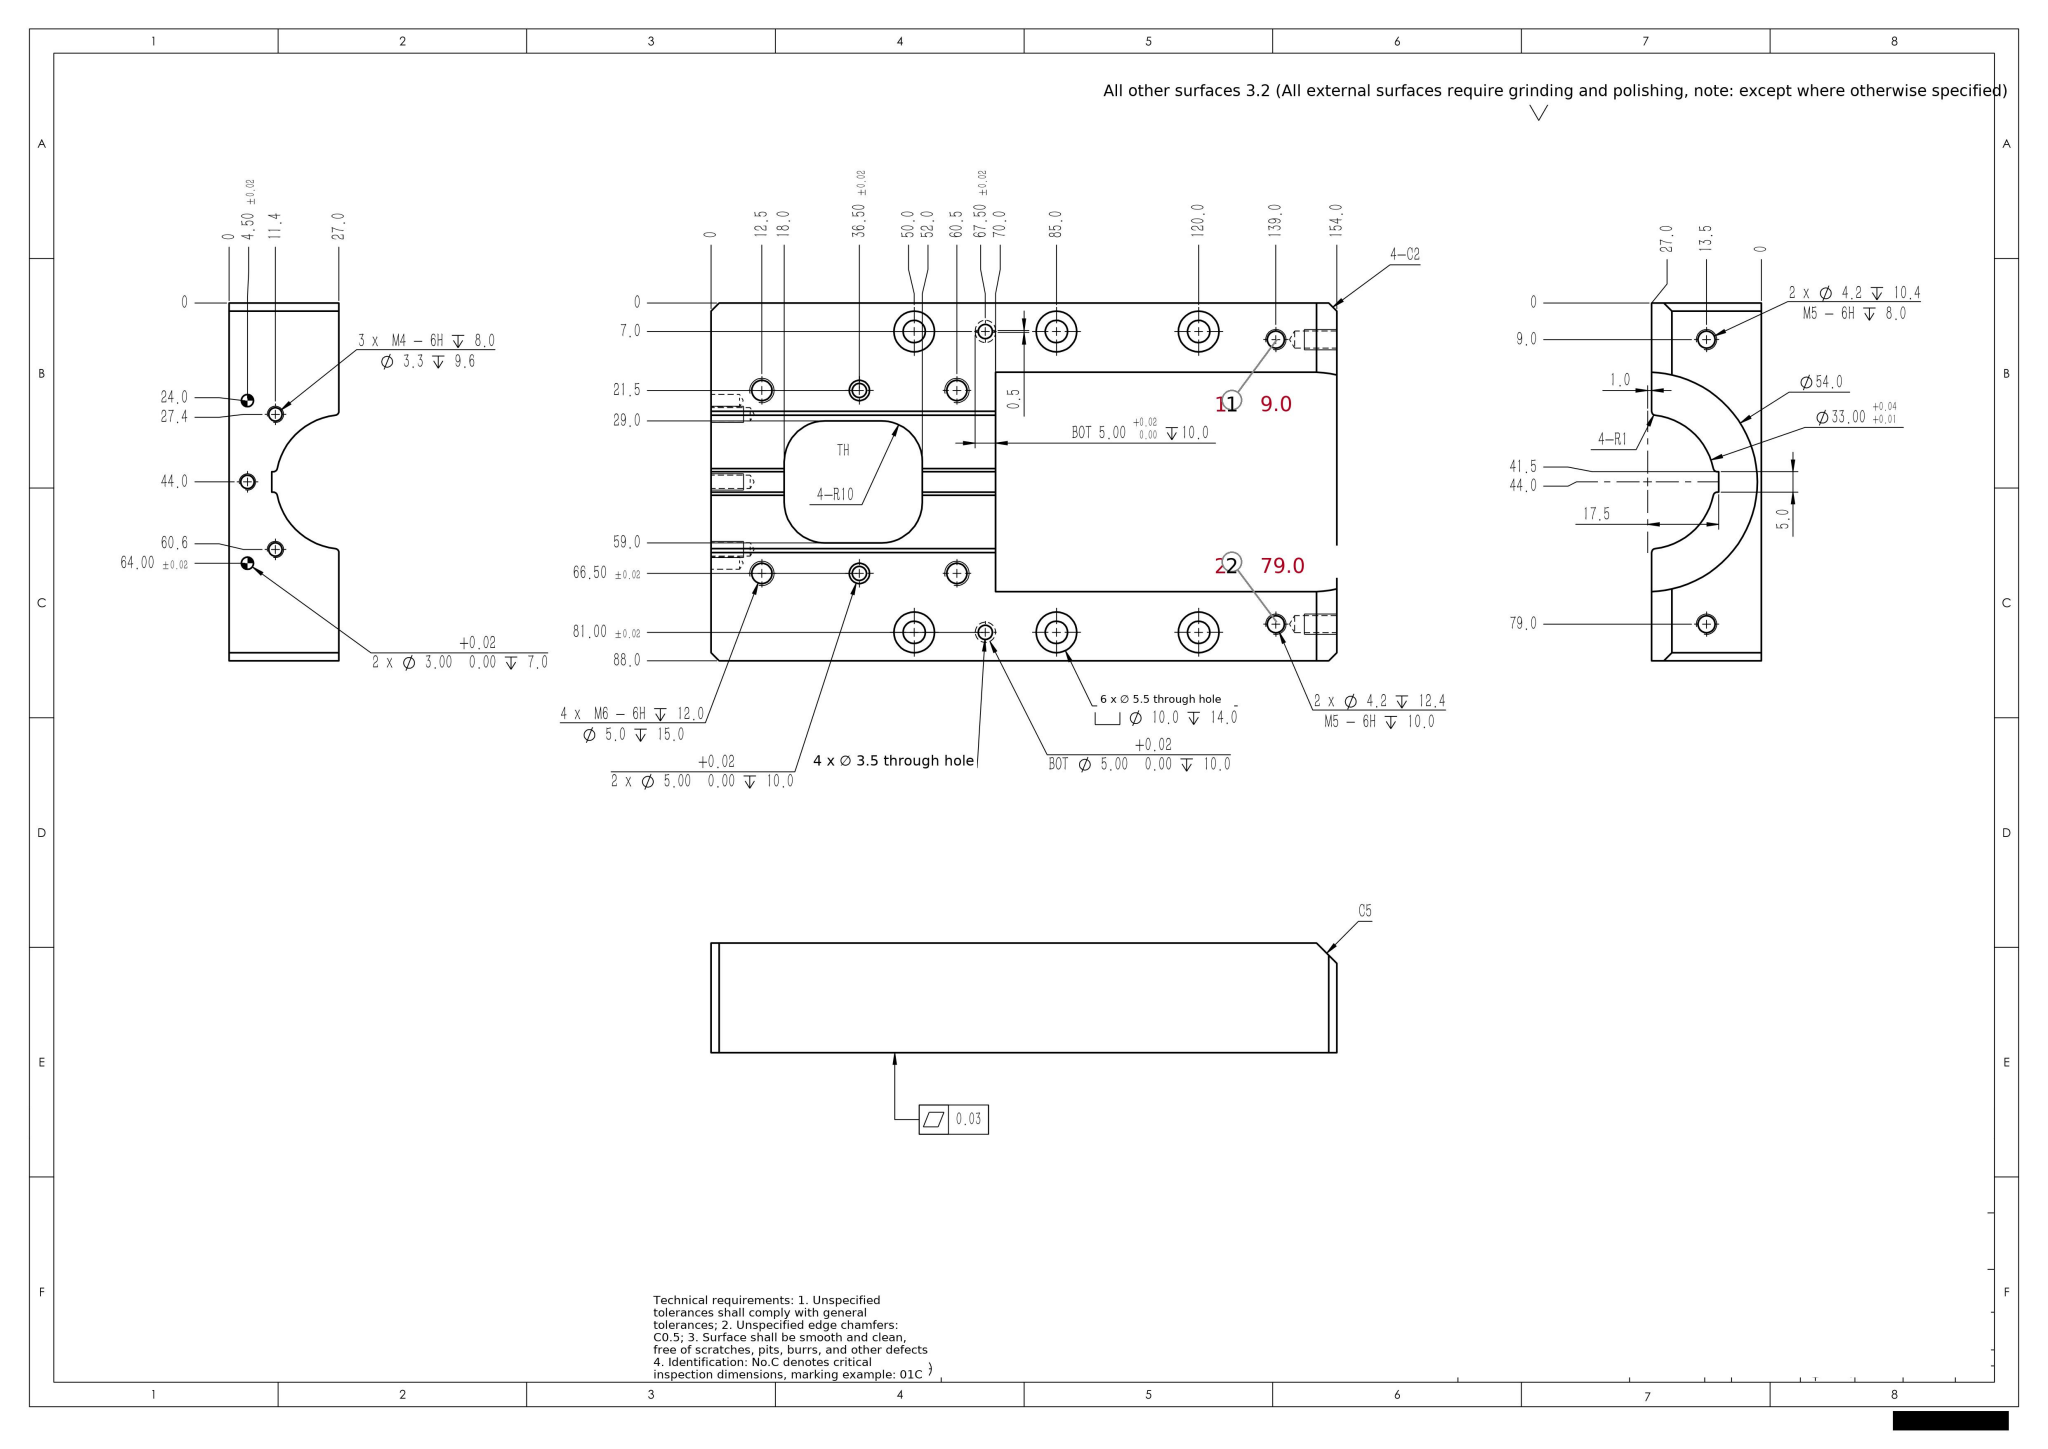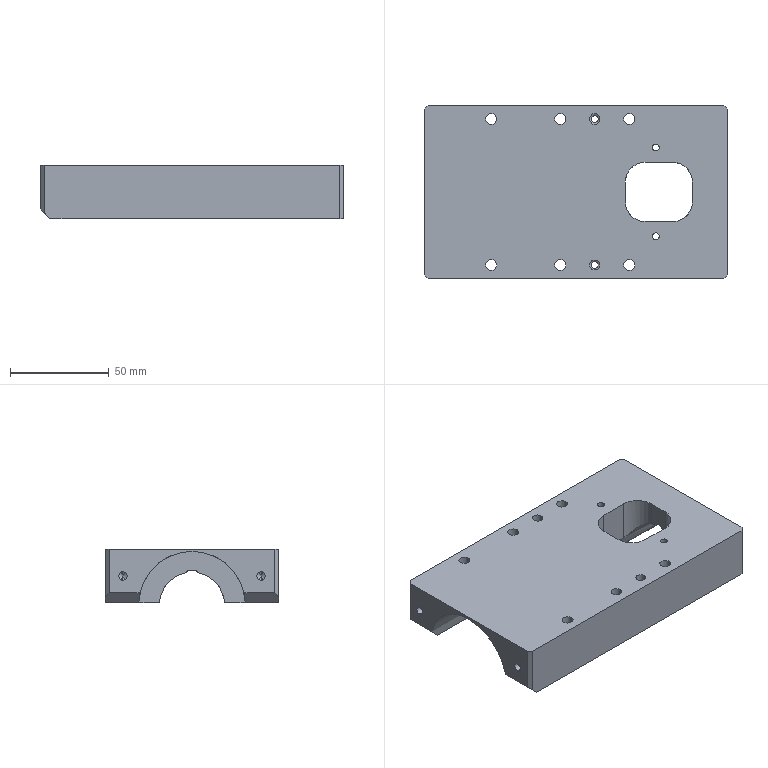Part | SolidWorks | mm | 1 solid | 148 faces | box 154 x 88 x 27 mm | volume 220663 mm3 | cylinder 80 | cone 34 | plane 34 | commonest cylinder face diameters 5 x16 10 x12 5.5 x12 4.2 x8 3.5 x8 3.3 x6 2 x6 3 x4